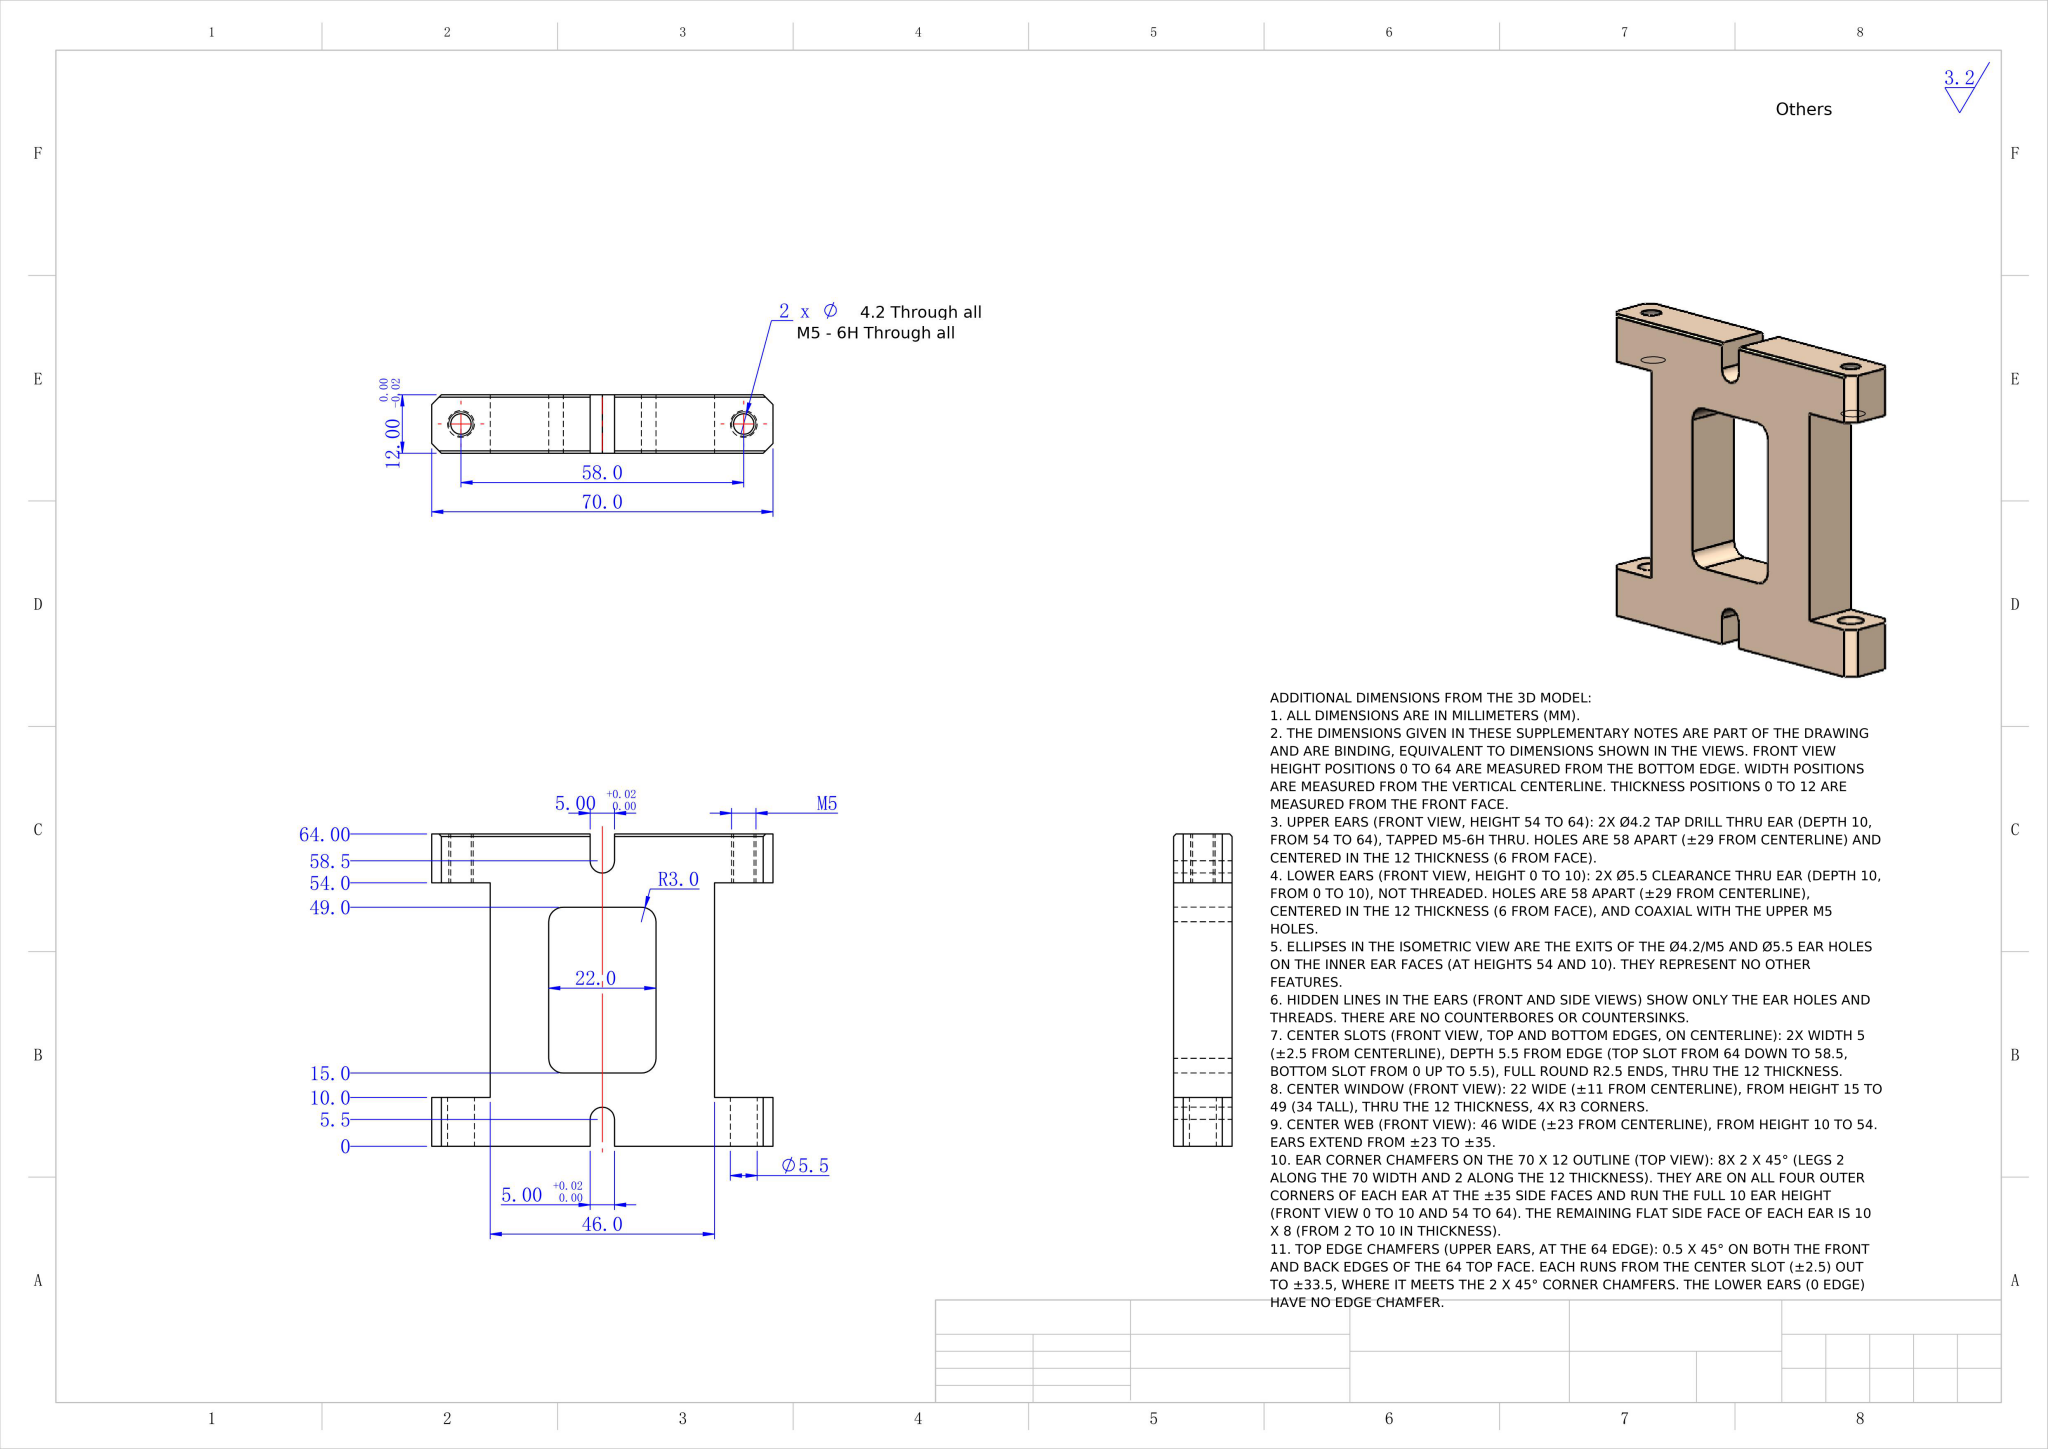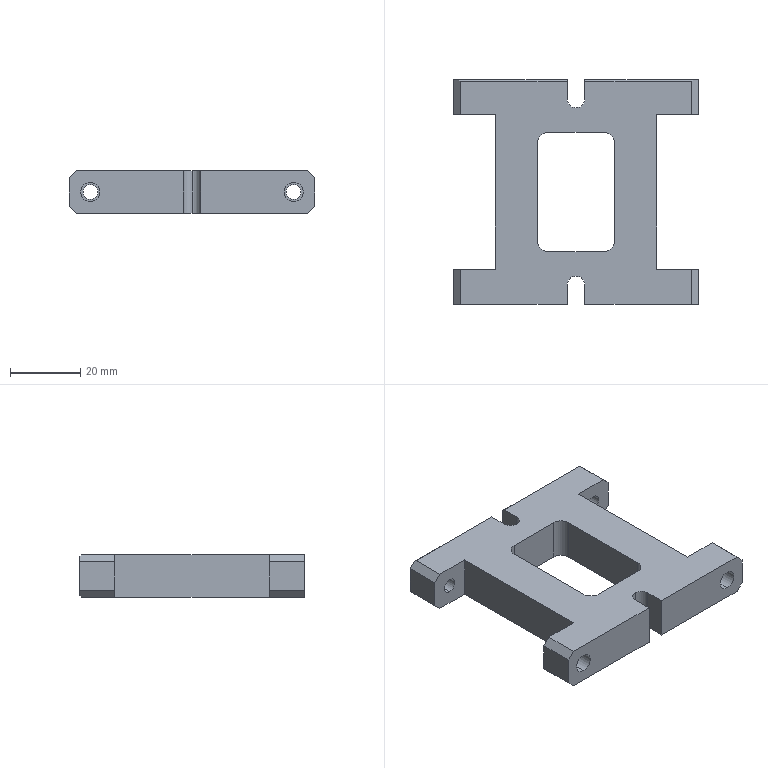Part | NX | mm | 1 solid | 52 faces | box 70 x 64 x 12 mm | volume 30382 mm3 | plane 36 | cylinder 16 | commonest cylinder face diameters 4.2 x4 5.5 x4 6 x4 5 x4